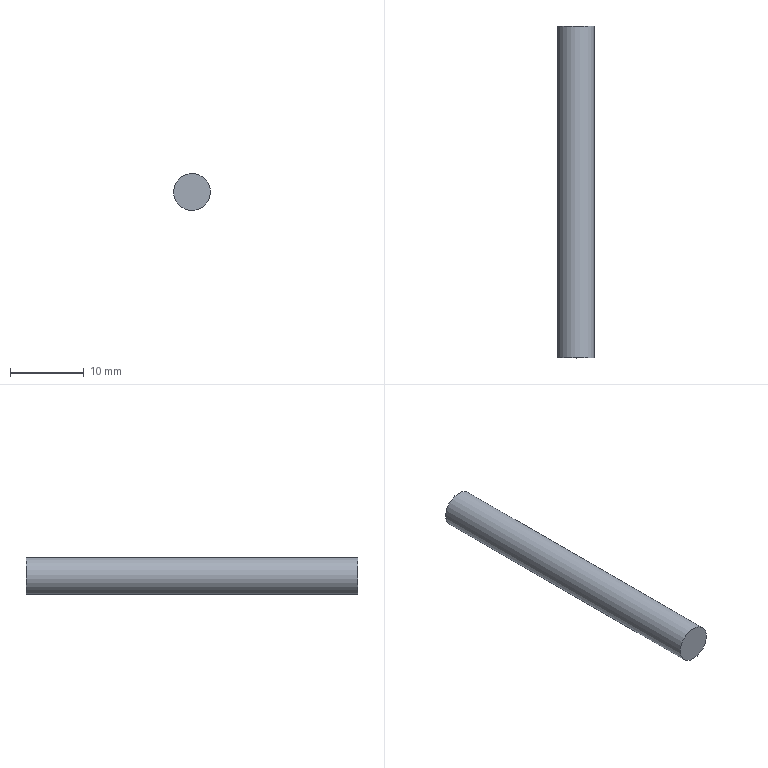Component | NX | PIN | 1 solid | 3 faces | box 5 x 45 x 5 mm | volume 884 mm3 | plane 2 | cylinder 1 | commonest cylinder face diameters 5 x1
STEP:
#1=CARTESIAN_POINT('',(0.,0.,0.));
#2=DIRECTION('',(0.,0.,1.));
#3=DIRECTION('',(1.,0.,0.));
#4=AXIS2_PLACEMENT_3D('',#1,#2,#3);
#5=CARTESIAN_POINT('',(2.598,22.5,109.741));
#6=VERTEX_POINT('',#5);
#7=CARTESIAN_POINT('',(0.1056,22.5,109.935));
#8=DIRECTION('',(0.,-1.,0.));
#9=DIRECTION('',(0.997,0.,-0.07746));
#10=AXIS2_PLACEMENT_3D('',#7,#8,#9);
#11=CIRCLE('',#10,2.5);
#12=CARTESIAN_POINT('',(0.1056,22.5,109.935));
#13=DIRECTION('',(0.,1.,0.));
#14=DIRECTION('',(0.07746,0.,0.997));
#15=AXIS2_PLACEMENT_3D('',#12,#13,#14);
#16=CYLINDRICAL_SURFACE('',#15,2.5);
#17=CARTESIAN_POINT('',(7.854,0.));
#18=DIRECTION('',(-1.,0.));
#19=VECTOR('',#18,1.);
#20=LINE('',#17,#19);
#21=(GEOMETRIC_REPRESENTATION_CONTEXT(2)PARAMETRIC_REPRESENTATION_CONTEXT()REPRESENTATION_CONTEXT('',''));
#22=DEFINITIONAL_REPRESENTATION('',(#20),#21);
#23=PCURVE('',#16,#22);
#24=CARTESIAN_POINT('',(0.1056,22.5,109.935));
#25=DIRECTION('',(0.,-1.,0.));
#26=DIRECTION('',(-0.07746,0.,-0.997));
#27=AXIS2_PLACEMENT_3D('',#24,#25,#26);
#28=PLANE('',#27);
#29=CARTESIAN_POINT('',(0.,0.));
#30=DIRECTION('',(-0.,1.));
#31=AXIS2_PLACEMENT_2D('',#29,#30);
#32=CIRCLE('',#31,2.5);
#33=(GEOMETRIC_REPRESENTATION_CONTEXT(2)PARAMETRIC_REPRESENTATION_CONTEXT()REPRESENTATION_CONTEXT('',''));
#34=DEFINITIONAL_REPRESENTATION('',(#32),#33);
#35=PCURVE('',#28,#34);
#36=SURFACE_CURVE('',#11,(#23,#35),.PCURVE_S1.);
#37=EDGE_CURVE('',#6,#6,#36,.T.);
#38=ORIENTED_EDGE('',*,*,#37,.F.);
#39=CARTESIAN_POINT('',(2.598,67.5,109.741));
#40=VERTEX_POINT('',#39);
#41=CARTESIAN_POINT('',(2.598,22.5,109.741));
#42=CARTESIAN_POINT('',(2.598,67.5,109.741));
#43=B_SPLINE_CURVE_WITH_KNOTS('',1,(#41,#42),.UNSPECIFIED.,.F.,.F.,(2,2),(0.,45.),.PIECEWISE_BEZIER_KNOTS.);
#44=CARTESIAN_POINT('',(7.854,0.));
#45=DIRECTION('',(0.,1.));
#46=VECTOR('',#45,1.);
#47=LINE('',#44,#46);
#48=(GEOMETRIC_REPRESENTATION_CONTEXT(2)PARAMETRIC_REPRESENTATION_CONTEXT()REPRESENTATION_CONTEXT('',''));
#49=DEFINITIONAL_REPRESENTATION('',(#47),#48);
#50=PCURVE('',#16,#49);
#51=CARTESIAN_POINT('',(1.571,0.));
#52=DIRECTION('',(0.,1.));
#53=VECTOR('',#52,1.);
#54=LINE('',#51,#53);
#55=(GEOMETRIC_REPRESENTATION_CONTEXT(2)PARAMETRIC_REPRESENTATION_CONTEXT()REPRESENTATION_CONTEXT('',''));
#56=DEFINITIONAL_REPRESENTATION('',(#54),#55);
#57=PCURVE('',#16,#56);
#58=SEAM_CURVE('',#43,(#50,#57),.PCURVE_S1.);
#59=EDGE_CURVE('',#6,#40,#58,.T.);
#60=ORIENTED_EDGE('',*,*,#59,.T.);
#61=CARTESIAN_POINT('',(0.1056,67.5,109.935));
#62=DIRECTION('',(0.,-1.,0.));
#63=DIRECTION('',(0.997,0.,-0.07746));
#64=AXIS2_PLACEMENT_3D('',#61,#62,#63);
#65=CIRCLE('',#64,2.5);
#66=CARTESIAN_POINT('',(7.854,45.));
#67=DIRECTION('',(-1.,0.));
#68=VECTOR('',#67,1.);
#69=LINE('',#66,#68);
#70=(GEOMETRIC_REPRESENTATION_CONTEXT(2)PARAMETRIC_REPRESENTATION_CONTEXT()REPRESENTATION_CONTEXT('',''));
#71=DEFINITIONAL_REPRESENTATION('',(#69),#70);
#72=PCURVE('',#16,#71);
#73=CARTESIAN_POINT('',(0.1056,67.5,109.935));
#74=DIRECTION('',(0.,-1.,0.));
#75=DIRECTION('',(-0.07746,0.,-0.997));
#76=AXIS2_PLACEMENT_3D('',#73,#74,#75);
#77=PLANE('',#76);
#78=CARTESIAN_POINT('',(0.,0.));
#79=DIRECTION('',(-0.,1.));
#80=AXIS2_PLACEMENT_2D('',#78,#79);
#81=CIRCLE('',#80,2.5);
#82=(GEOMETRIC_REPRESENTATION_CONTEXT(2)PARAMETRIC_REPRESENTATION_CONTEXT()REPRESENTATION_CONTEXT('',''));
#83=DEFINITIONAL_REPRESENTATION('',(#81),#82);
#84=PCURVE('',#77,#83);
#85=SURFACE_CURVE('',#65,(#72,#84),.PCURVE_S1.);
#86=EDGE_CURVE('',#40,#40,#85,.T.);
#87=ORIENTED_EDGE('',*,*,#86,.T.);
#88=ORIENTED_EDGE('',*,*,#59,.F.);
#89=EDGE_LOOP('',(#38,#60,#87,#88));
#90=FACE_BOUND('',#89,.T.);
#91=ADVANCED_FACE('',(#90),#16,.T.);
#92=ORIENTED_EDGE('',*,*,#37,.T.);
#93=EDGE_LOOP('',(#92));
#94=FACE_BOUND('',#93,.T.);
#95=ADVANCED_FACE('',(#94),#28,.T.);
#96=ORIENTED_EDGE('',*,*,#86,.F.);
#97=EDGE_LOOP('',(#96));
#98=FACE_BOUND('',#97,.T.);
#99=ADVANCED_FACE('',(#98),#77,.F.);
#100=CLOSED_SHELL('',(#91,#95,#99));
#101=MANIFOLD_SOLID_BREP('',#100);
#102=(LENGTH_UNIT()NAMED_UNIT(*)SI_UNIT(.MILLI.,.METRE.));
#103=UNCERTAINTY_MEASURE_WITH_UNIT(LENGTH_MEASURE(0.00001),#102,'','');
#104=(NAMED_UNIT(*)PLANE_ANGLE_UNIT()SI_UNIT($,.RADIAN.));
#105=(NAMED_UNIT(*)SI_UNIT($,.STERADIAN.)SOLID_ANGLE_UNIT());
#106=(GEOMETRIC_REPRESENTATION_CONTEXT(3)GLOBAL_UNCERTAINTY_ASSIGNED_CONTEXT((#103))GLOBAL_UNIT_ASSIGNED_CONTEXT((#102,#104,#105))REPRESENTATION_CONTEXT('',''));
#107=ADVANCED_BREP_SHAPE_REPRESENTATION('',(#4,#101),#106);